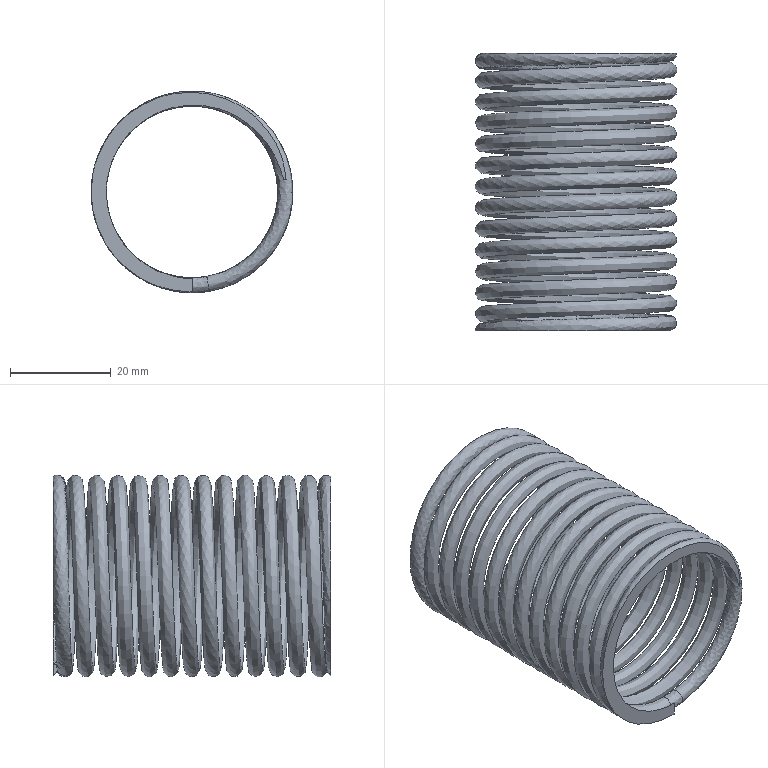Component | NX | COMP_SPRING | 1 solid | 9 faces | volume 10969 mm3 | spline 5 | plane 4